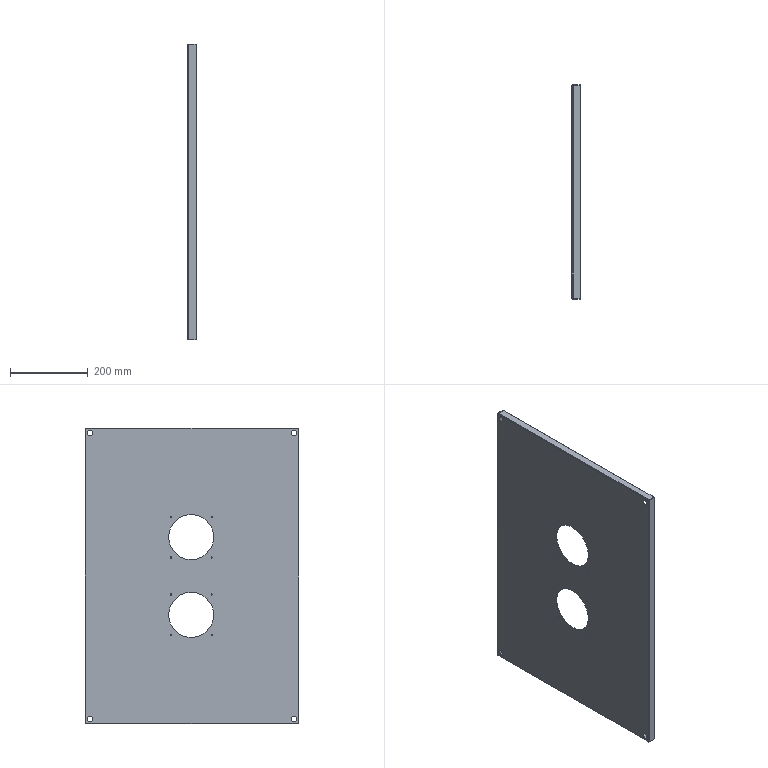Component | SolidWorks | TopCoverPlatePG50-102A-1 | 1 solid | 78 faces | volume 670966 mm3 | plane 42 | cylinder 36 | commonest cylinder face diameters 3.2 x16 14 x8 116 x4 3.3 x4 0.3 x4 | material AISI 1045 Steel, cold drawn